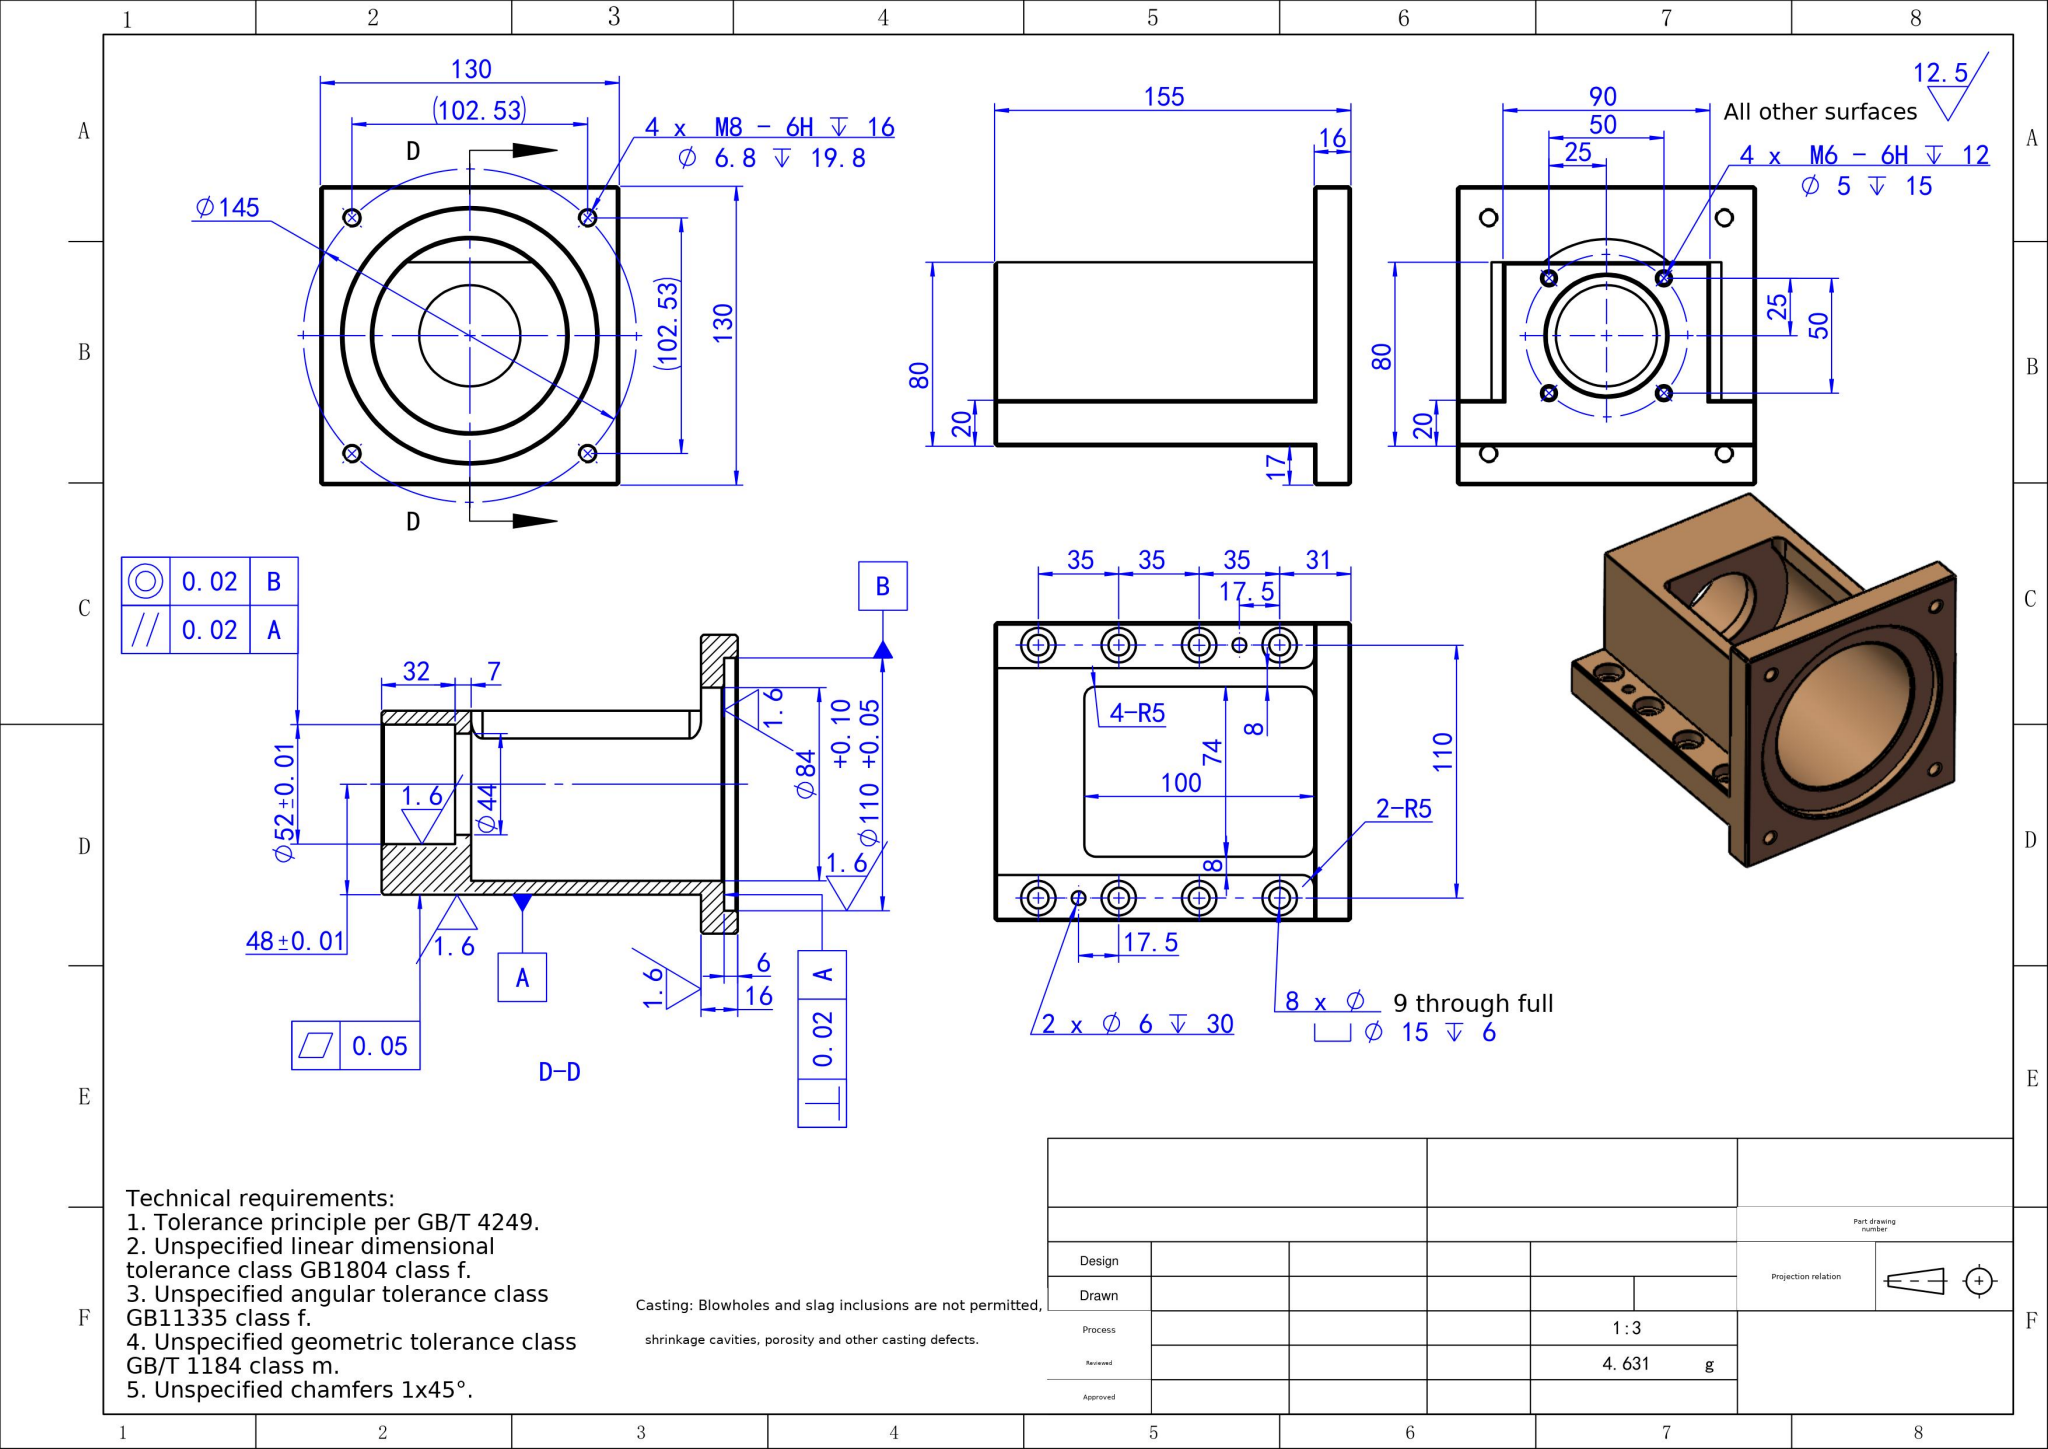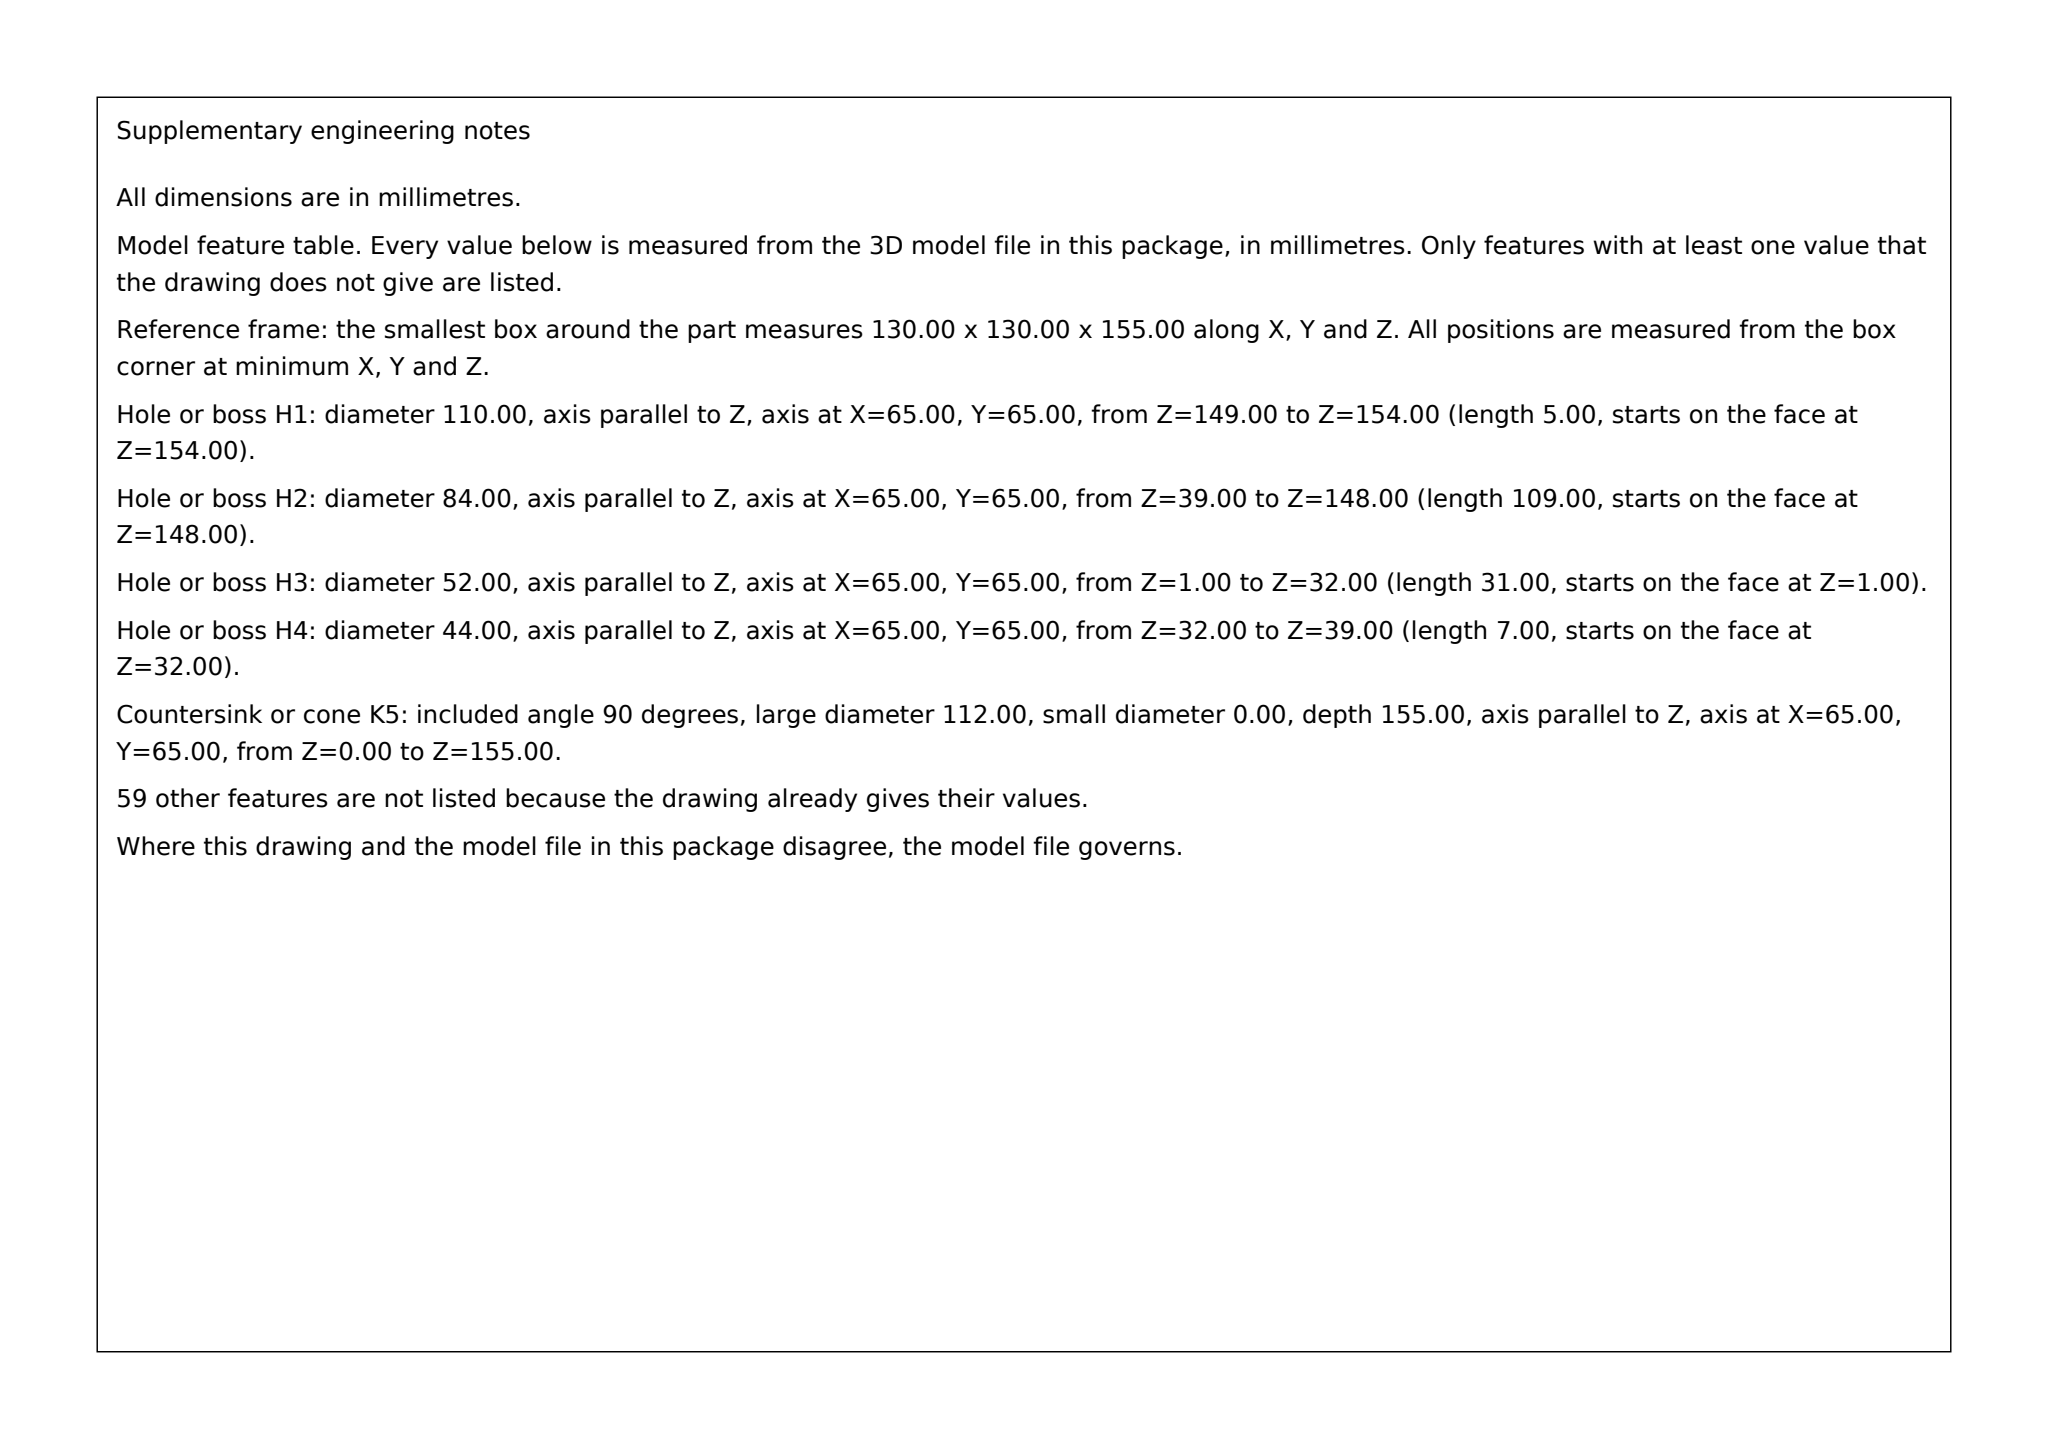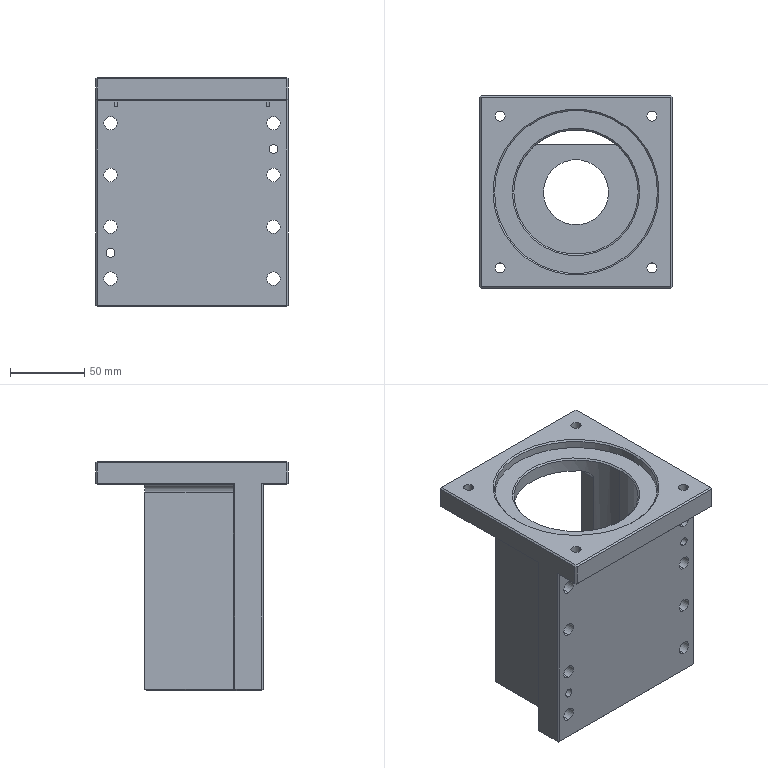Part | SolidWorks | mm | 1 solid | 155 faces | box 130 x 130 x 155 mm | volume 643199 mm3 | cylinder 66 | plane 65 | cone 24 | commonest cylinder face diameters 15 x16 9 x16 5 x8 6.8 x8 10 x6 6 x4 52 x2 110 x2